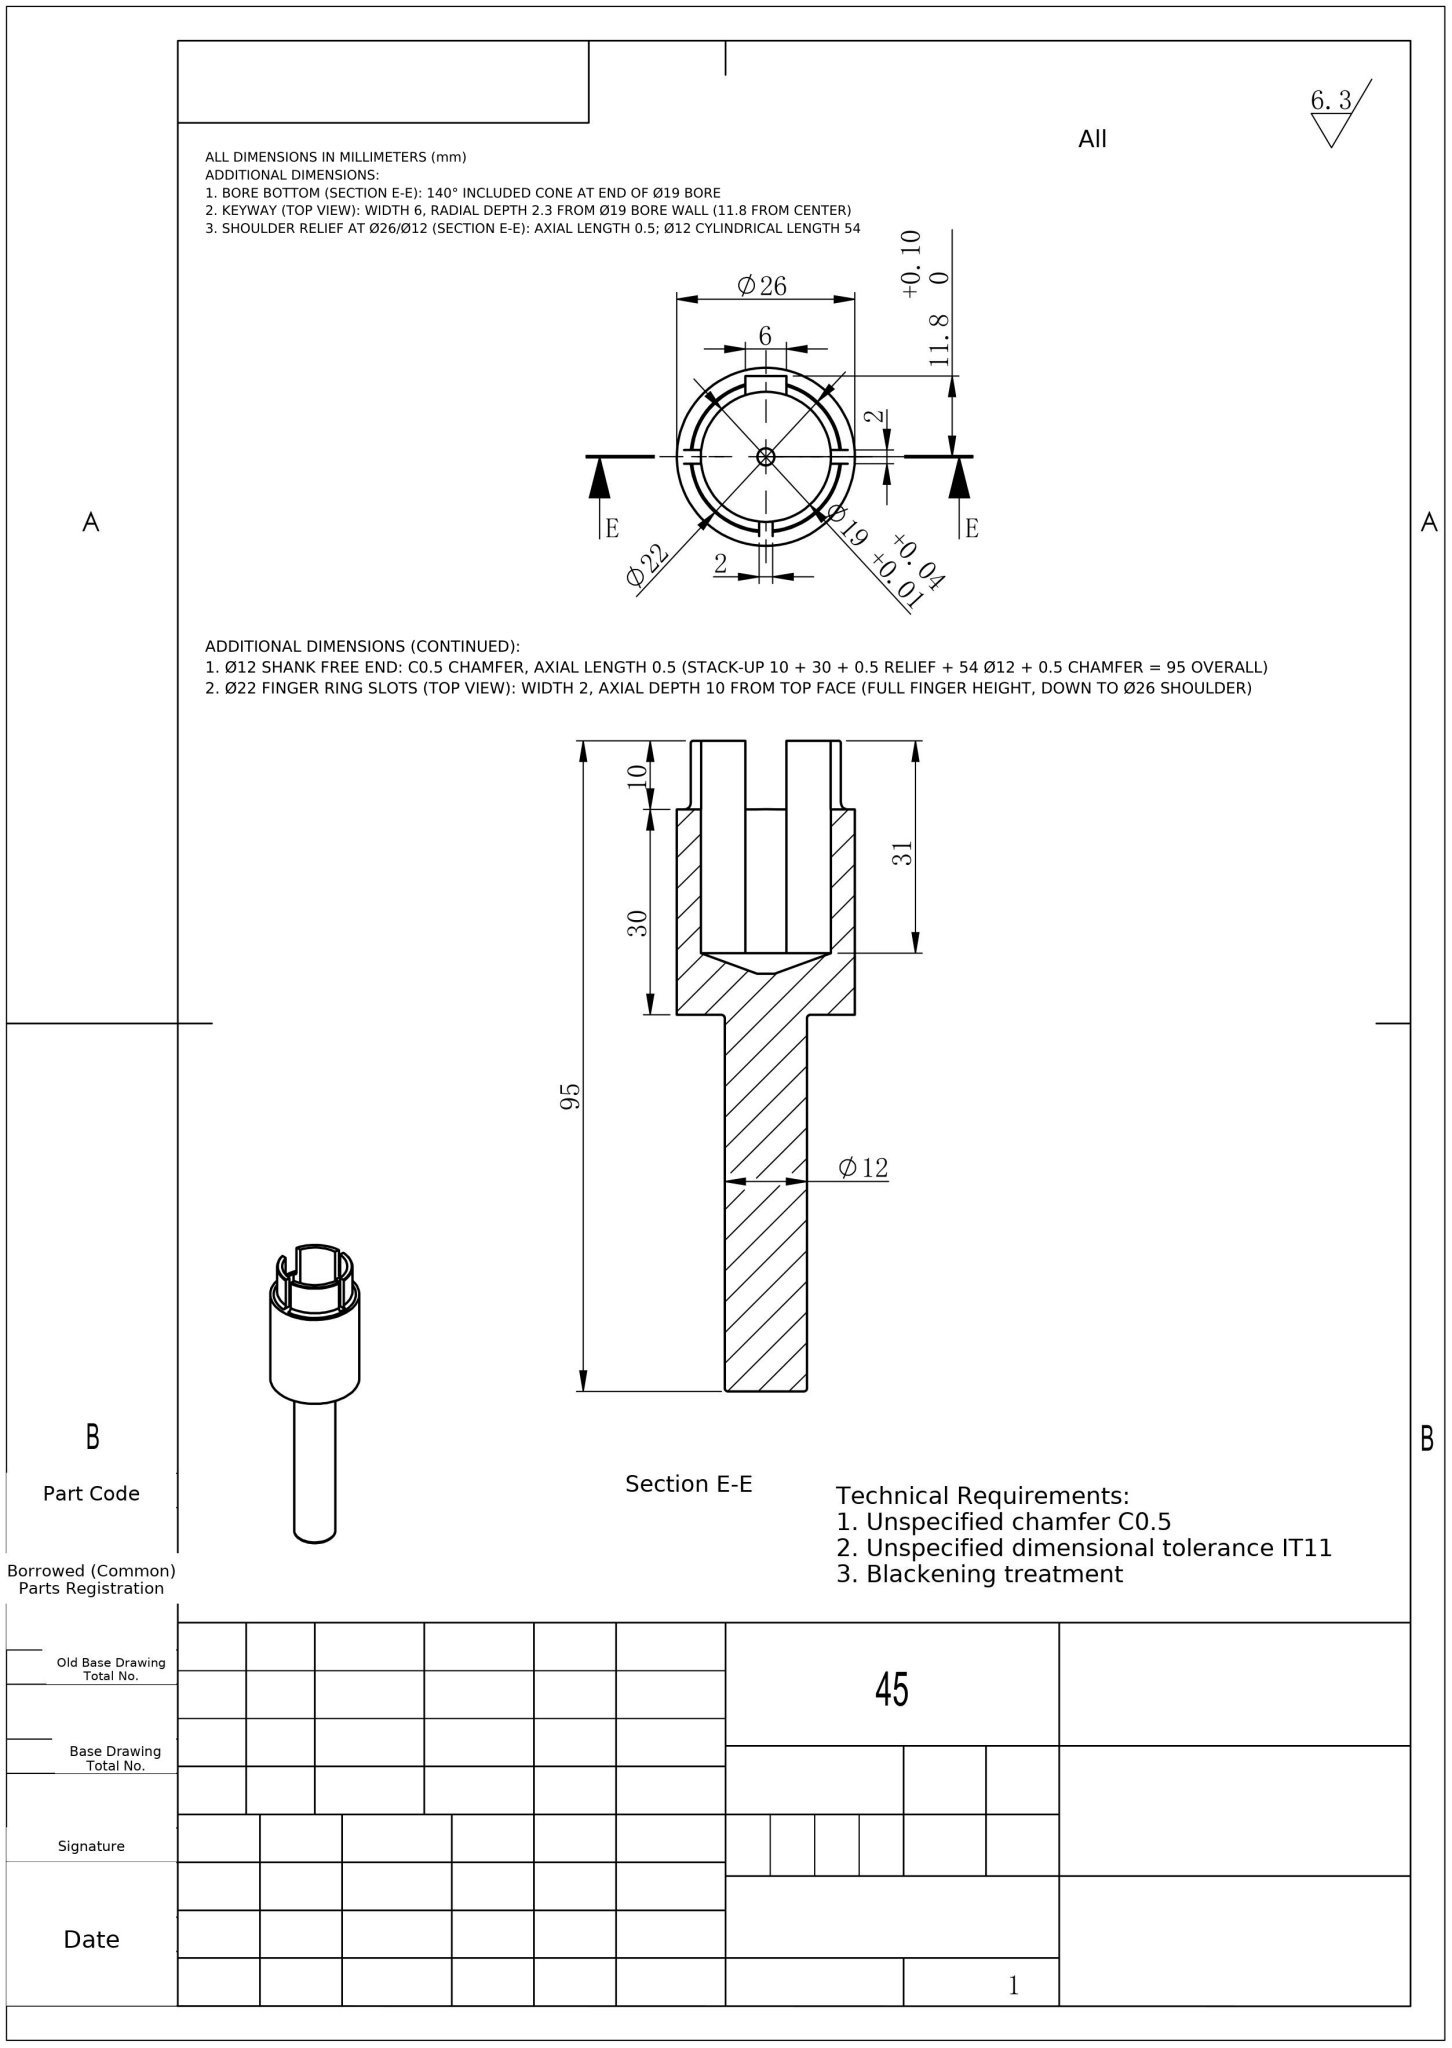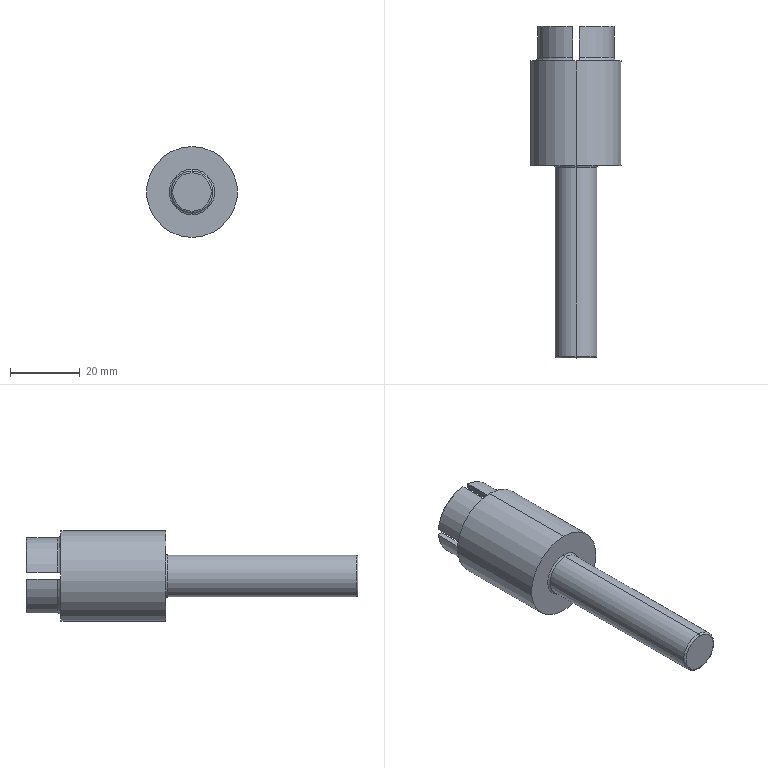Part | NX | mm | 1 solid | 45 faces | box 26 x 95 x 26 mm | volume 16354 mm3 | plane 20 | cylinder 10 | torus 9 | cone 6 | commonest cylinder face diameters 22 x4 12 x2 19 x2 26 x2